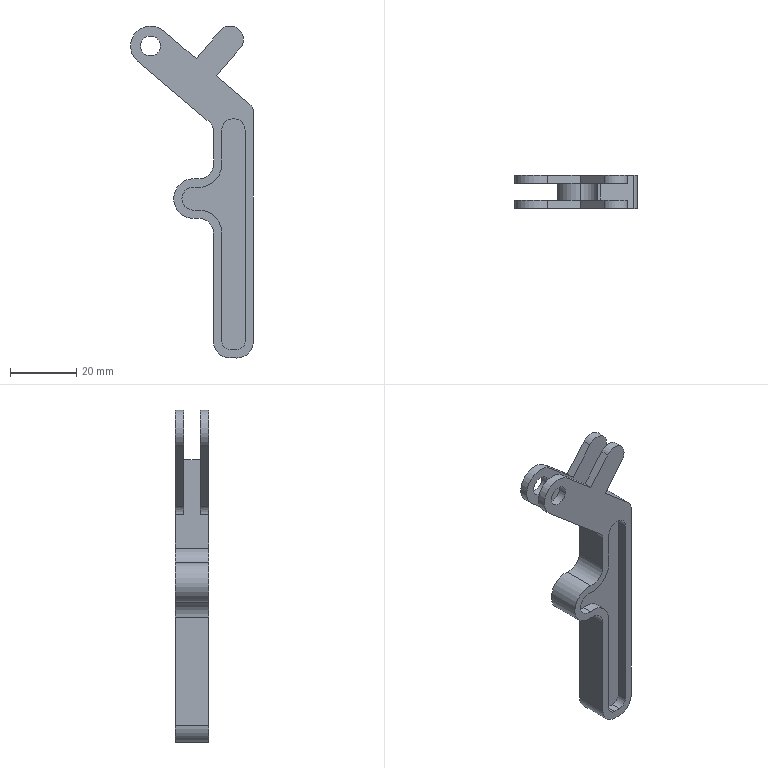Component | NX | HANDLE | 1 solid | 54 faces | volume 9669 mm3 | plane 28 | cylinder 26 | commonest cylinder face diameters 6 x5 7 x4 14 x4 5 x4 12 x3 8 x2 9 x2 10 x2